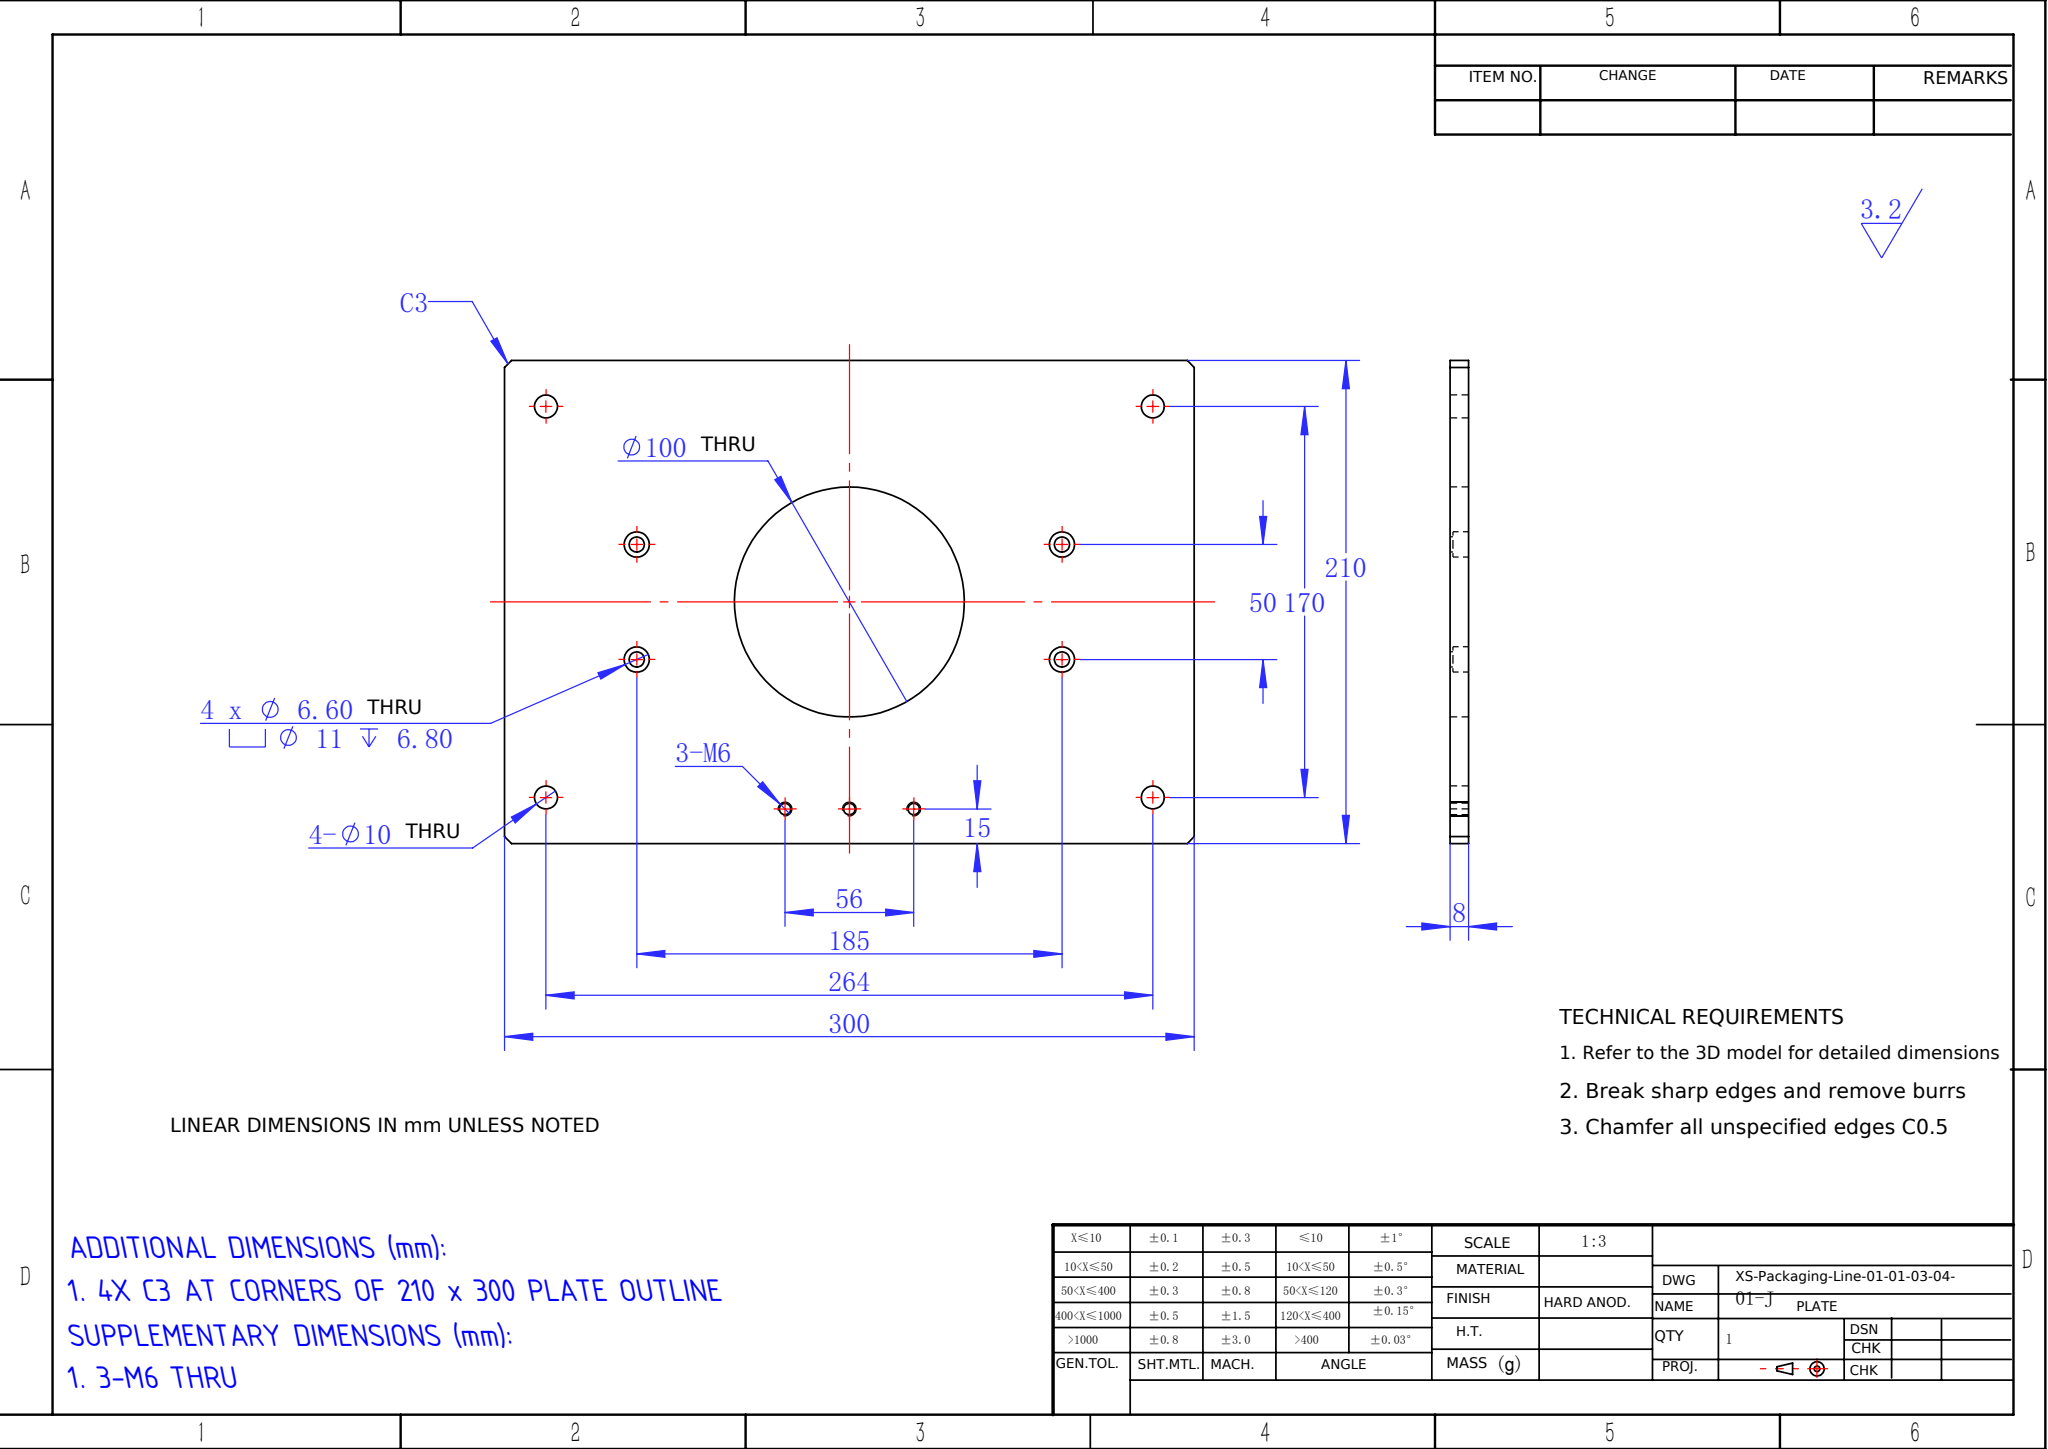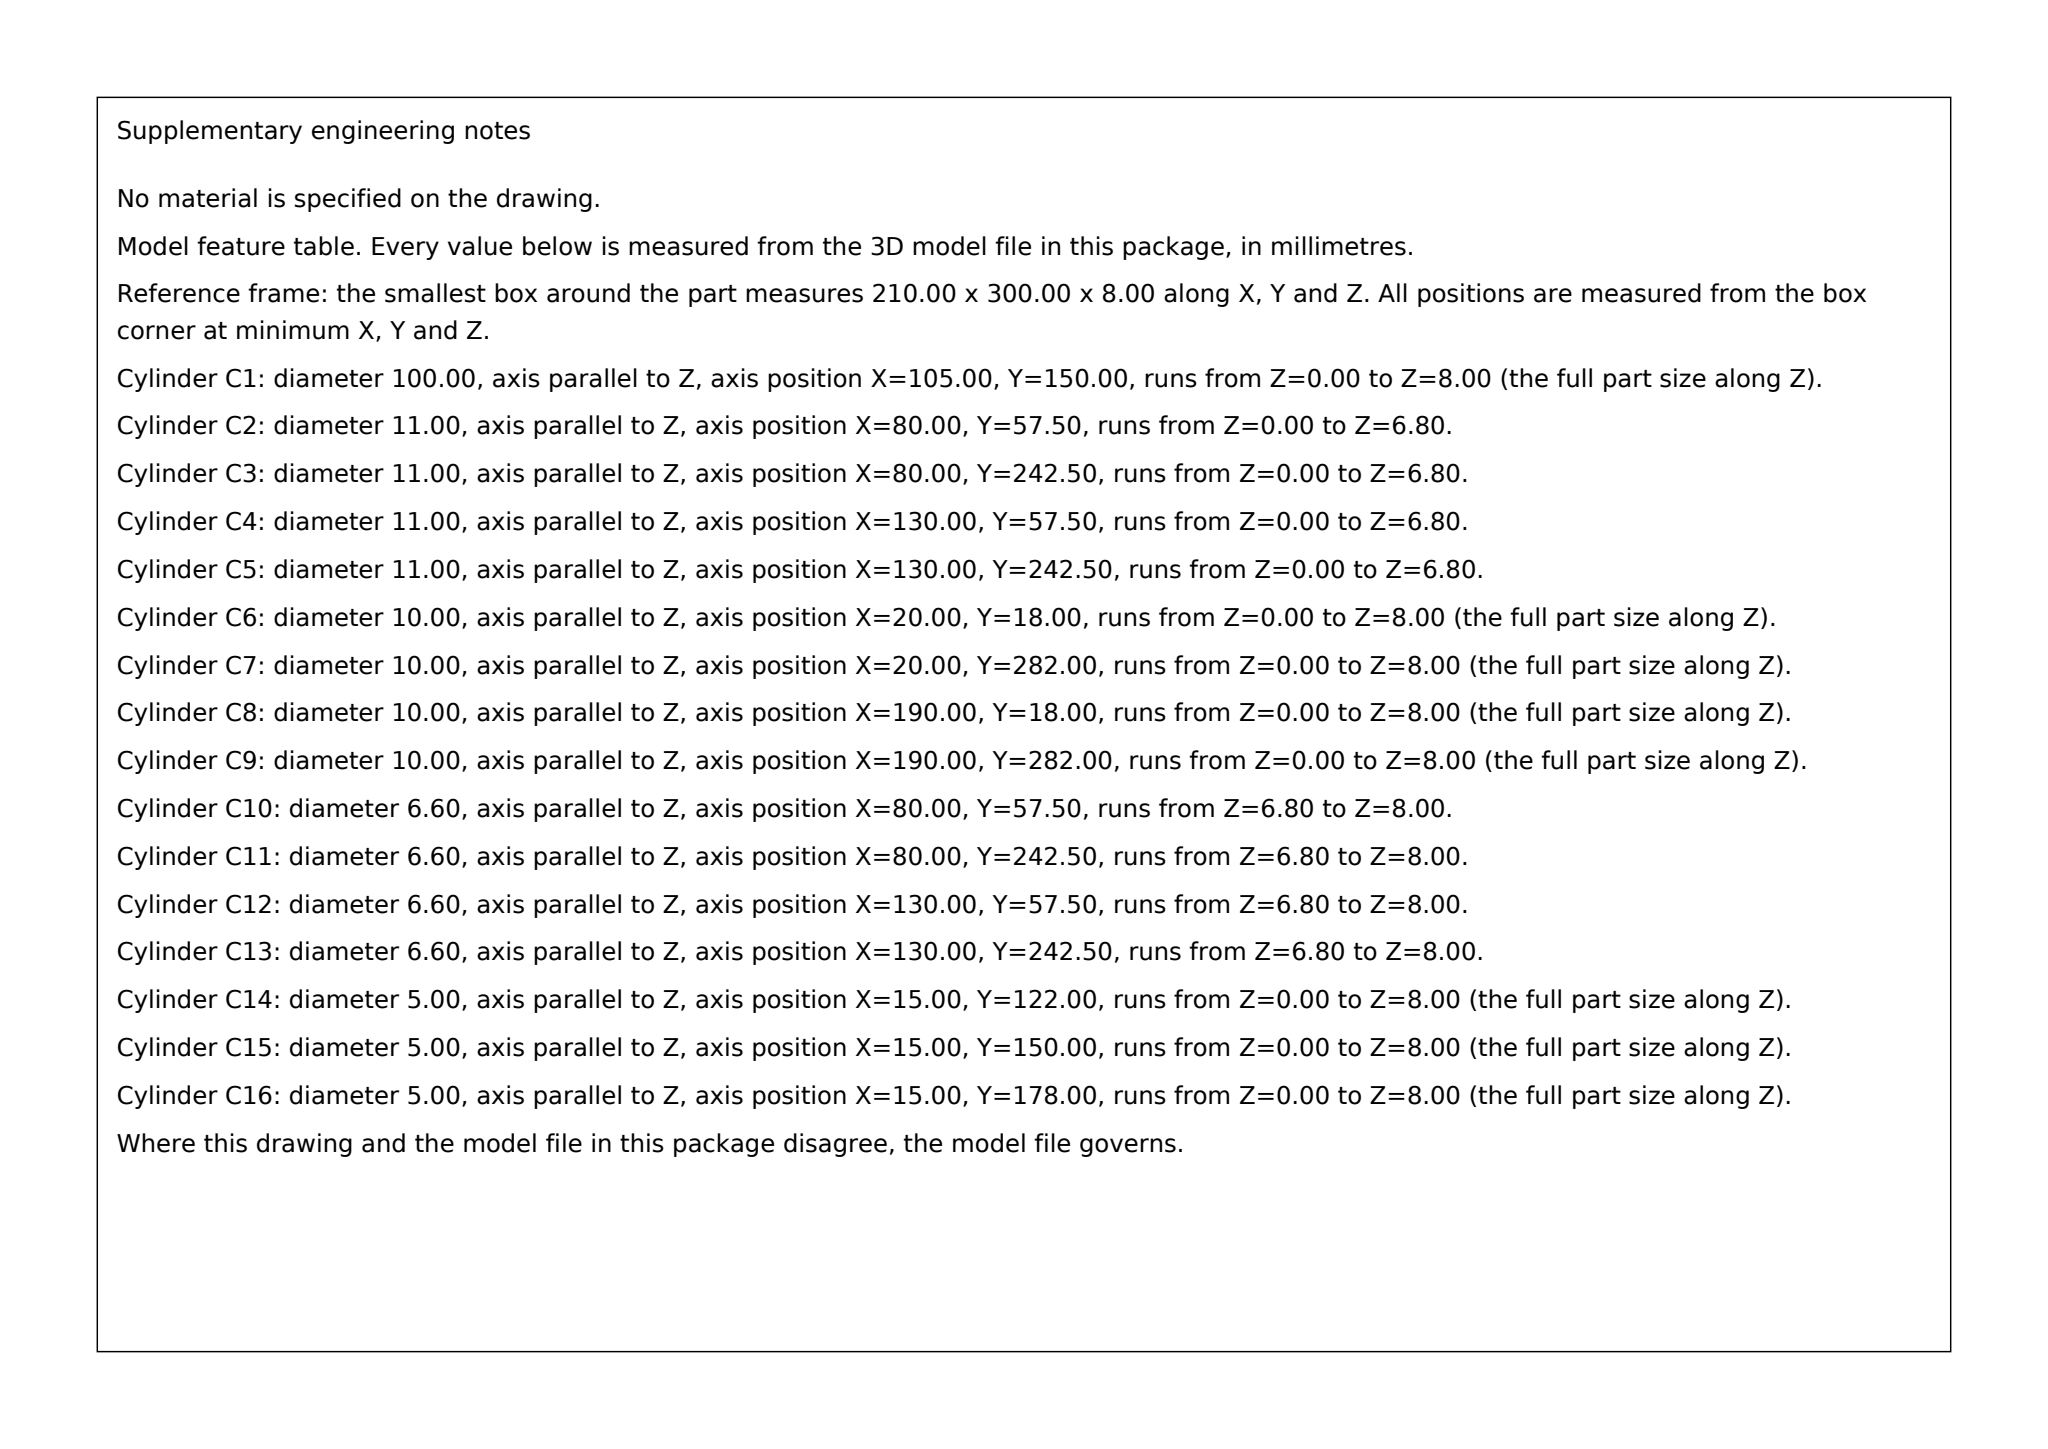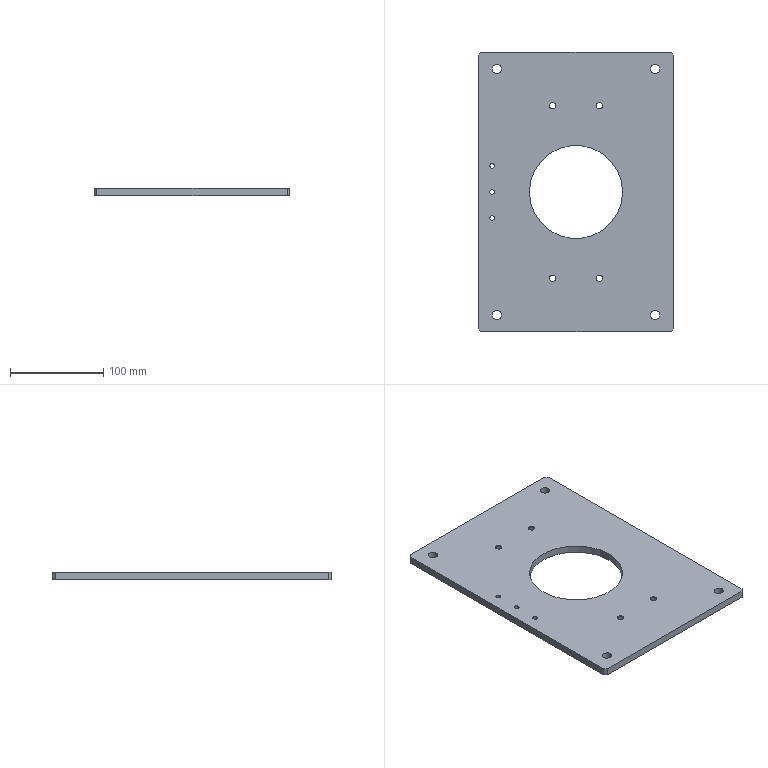Part | SolidWorks | mm | 1 solid | 46 faces | box 210 x 300 x 8 mm | volume 435291 mm3 | cylinder 32 | plane 14 | commonest cylinder face diameters 11 x8 6.6 x8 10 x8 5 x6 100 x2
build123d program:
from build123d import *

# Parameters (mm, degrees)
SKETCH1_W                                       = 210
SKETCH1_H                                       = 300
BOSS_EXTRUDE1_DEPTH                             = 8
SKETCH2_R                                       = 50
CUT_EXTRUDE1_DEPTH                              = 184.273
SKETCH3_R                                       = 5
CUT_EXTRUDE2_DEPTH                              = 184.273
CHAMFER1_SIZE                                   = 3
M6_HEX_SOCKET_HEAD_CAP_SCREW_CBORE1_D           = 6.6
M6_HEX_SOCKET_HEAD_CAP_SCREW_CBORE1_CBORE_D     = 11
M6_HEX_SOCKET_HEAD_CAP_SCREW_CBORE1_CBORE_DEPTH = 6.8
M6_TAPPED_HOLE1_D                               = 5
M6_TAPPED_HOLE2_D                               = 5
M6_TAPPED_HOLE2_DEPTH                           = 15
M6_TAPPED_HOLE2_TIP                             = 1.502


with BuildPart() as part:
    # Sketch1 → Boss-Extrude1 (new body)
    with BuildSketch(Plane.XY):
        Rectangle(SKETCH1_W, SKETCH1_H)
    extrude(amount=BOSS_EXTRUDE1_DEPTH)

    # Sketch2 → Cut-Extrude1 (cut, through all)
    with BuildSketch(Plane.XY.offset(8)):
        Circle(SKETCH2_R)
    extrude(amount=-CUT_EXTRUDE1_DEPTH, mode=Mode.SUBTRACT)

    # Sketch3 → Cut-Extrude2 (cut, through all)
    with BuildSketch(Plane.XY.offset(8)):
        with Locations((-85, 132)):
            Circle(SKETCH3_R)
        with Locations((85, 132)):
            Circle(SKETCH3_R)
        with Locations((-85, -132)):
            Circle(SKETCH3_R)
        with Locations((85, -132)):
            Circle(SKETCH3_R)
    extrude(amount=-CUT_EXTRUDE2_DEPTH, mode=Mode.SUBTRACT)

    # Chamfer1
    chamfer1_edges = [part.edges().sort_by_distance(p)[0] for p in [
        (105, -150, 4),
        (-105, -150, 4),
        (-105, 150, 4),
        (105, 150, 4),
    ]]
    chamfer(chamfer1_edges, length=CHAMFER1_SIZE)

    # M6 Hex Socket Head Cap Screw CBORE1 (through all)
    with Locations(Plane(origin=(0, 0, 0), x_dir=(-1, 0, 0), z_dir=(0, 0, -1))):
        with Locations((-25, 92.5), (25, 92.5), (-25, -92.5), (25, -92.5)):
            CounterBoreHole(M6_HEX_SOCKET_HEAD_CAP_SCREW_CBORE1_D / 2, M6_HEX_SOCKET_HEAD_CAP_SCREW_CBORE1_CBORE_D / 2, M6_HEX_SOCKET_HEAD_CAP_SCREW_CBORE1_CBORE_DEPTH)

    # M6 Tapped Hole1 (through all)
    with Locations(Plane.XY.offset(8)):
        with Locations((-90, 28), (-90, -28)):
            Hole(M6_TAPPED_HOLE1_D / 2)

    # M6 Tapped Hole2
    with Locations(Plane.XY.offset(8)):
        with Locations((-90, 0)):
            Hole(M6_TAPPED_HOLE2_D / 2, depth=M6_TAPPED_HOLE2_DEPTH)
            with Locations((0, 0, -(M6_TAPPED_HOLE2_DEPTH + M6_TAPPED_HOLE2_TIP / 2))):  # 118° drill point
                Cone(0, M6_TAPPED_HOLE2_D / 2, M6_TAPPED_HOLE2_TIP, mode=Mode.SUBTRACT)


solid = part.part